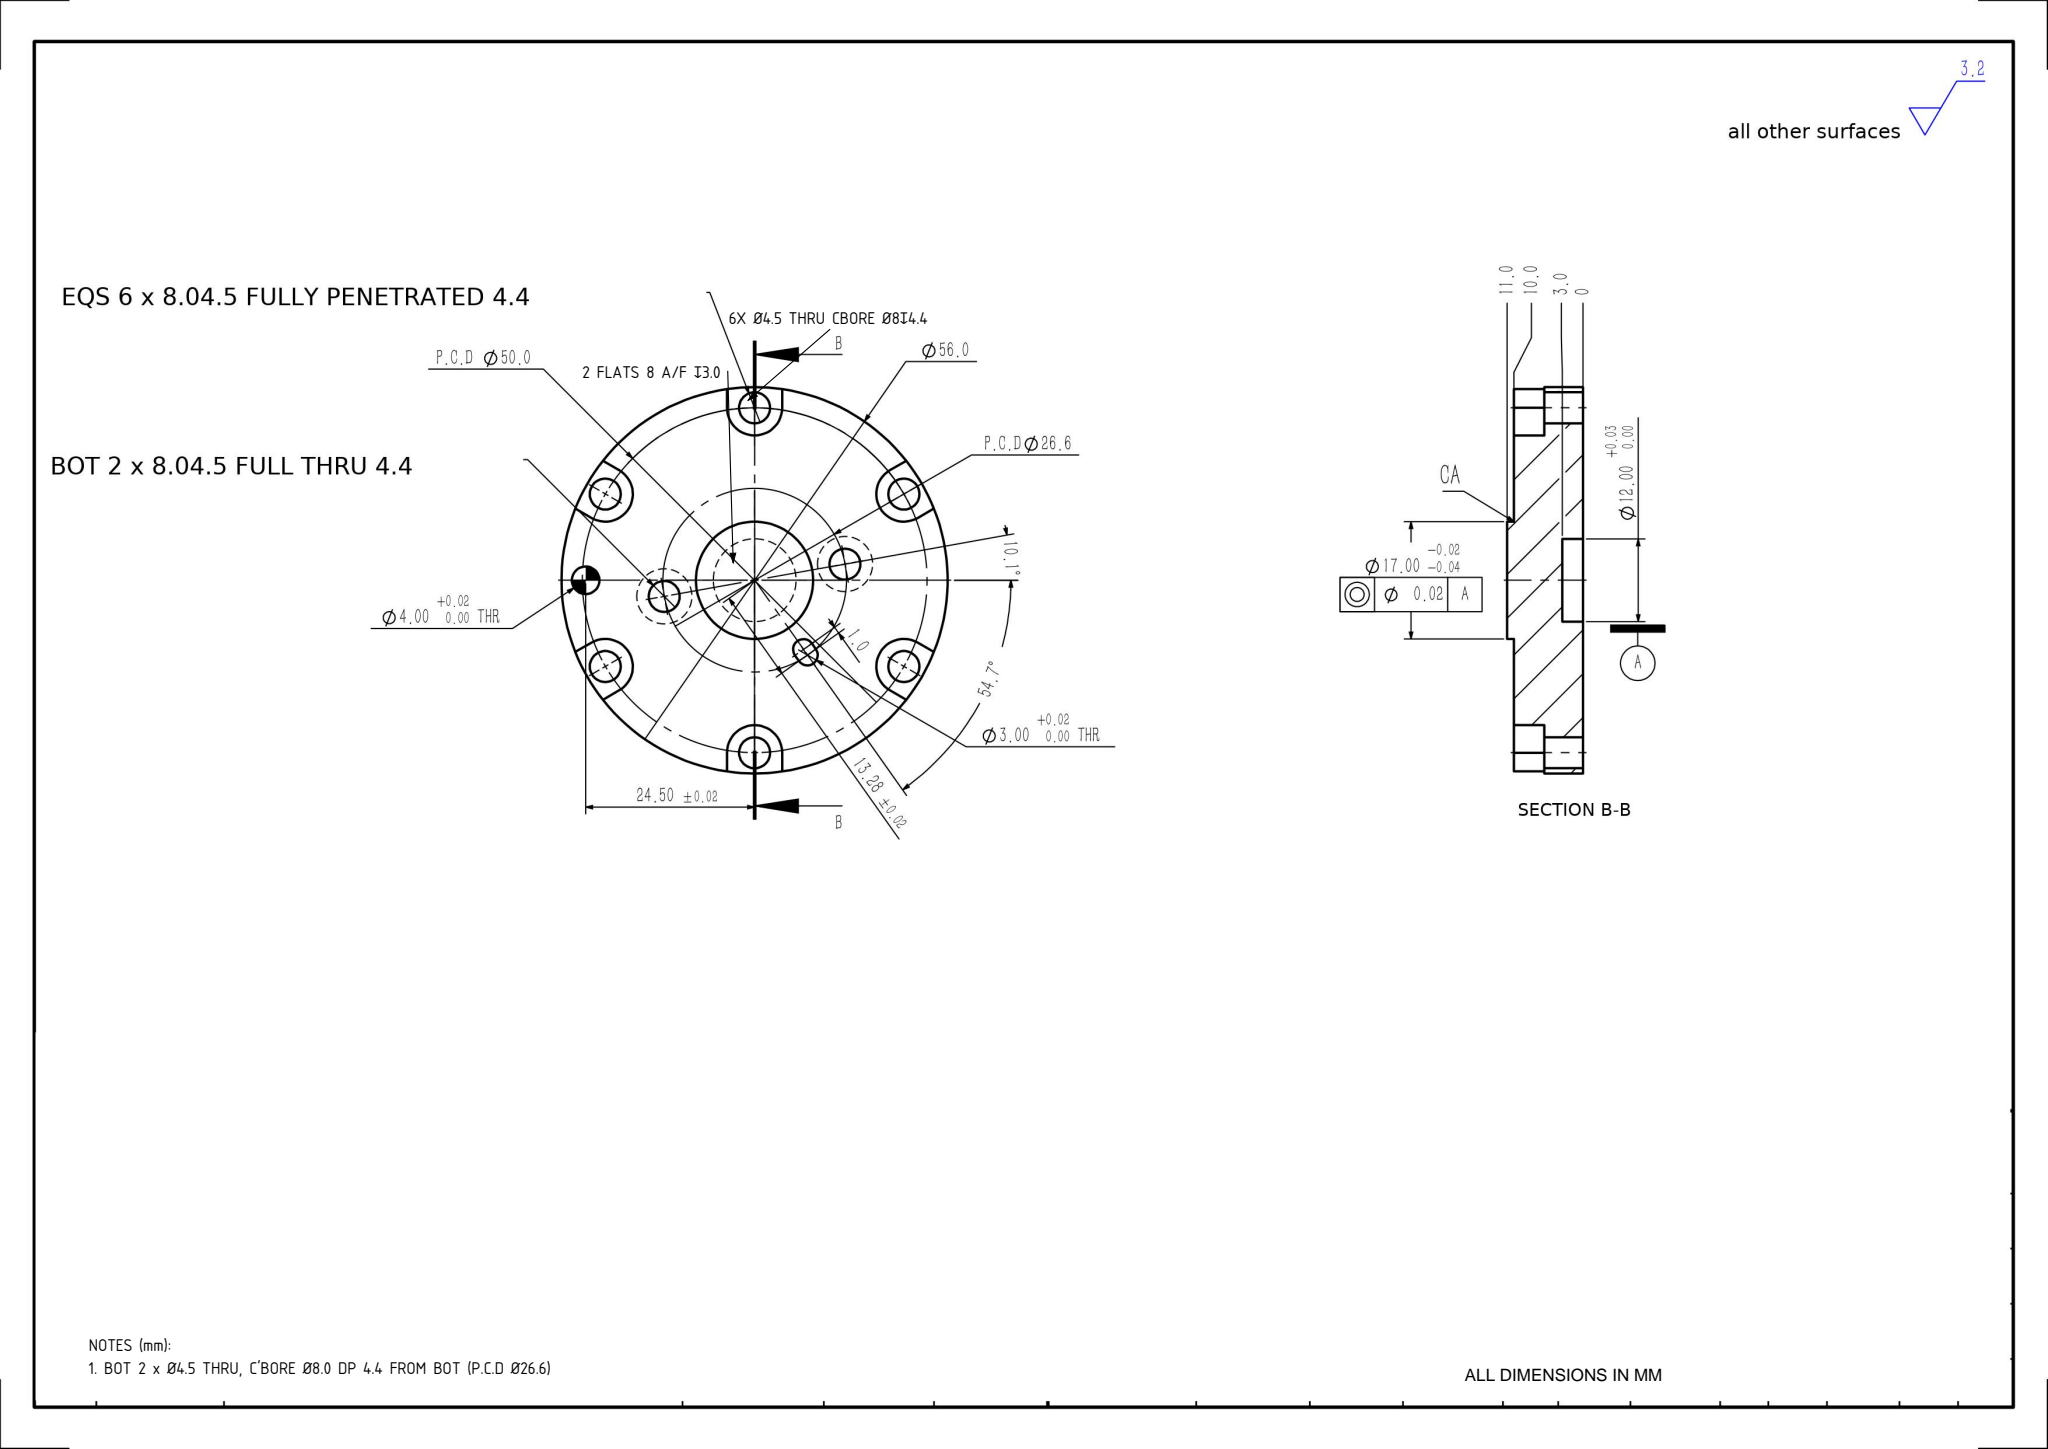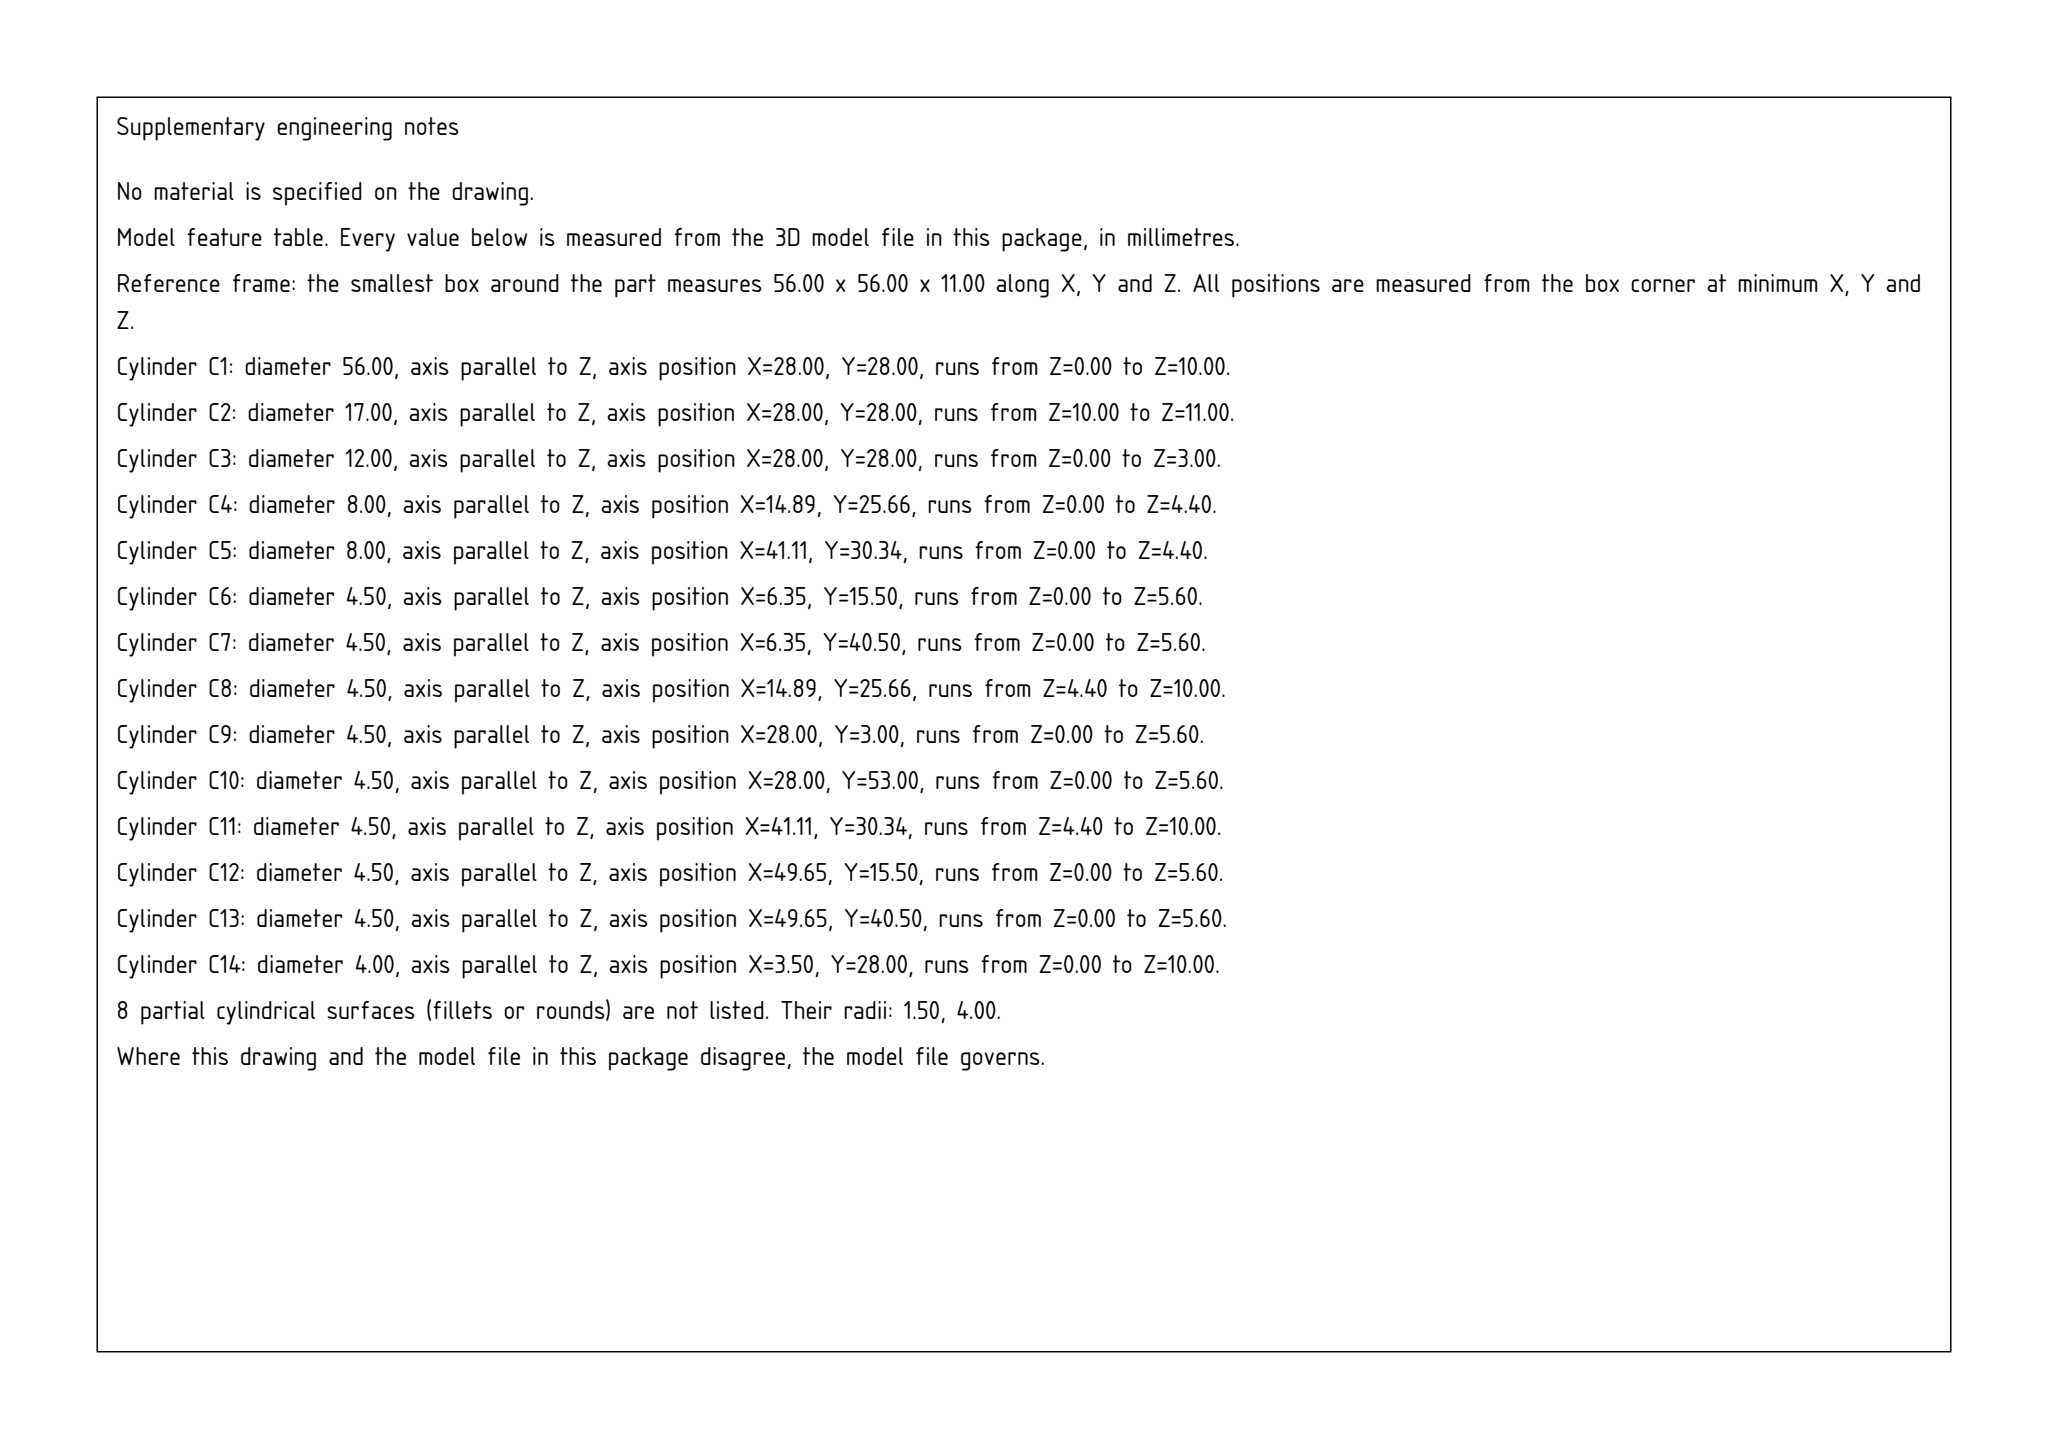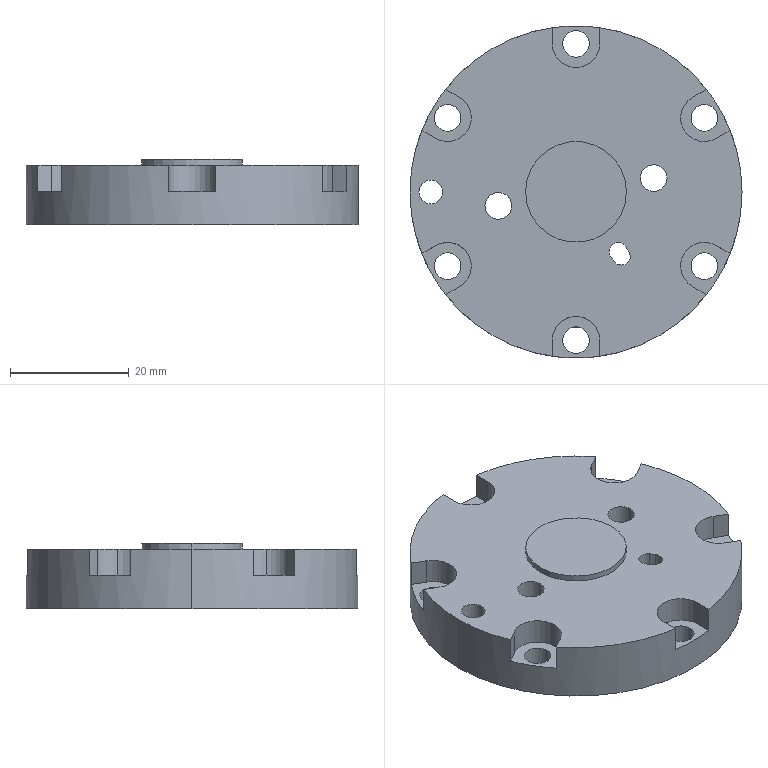Part | SolidWorks | mm | 1 solid | 65 faces | box 56 x 56 x 11 mm | volume 21860 mm3 | cylinder 39 | plane 26 | commonest cylinder face diameters 4.5 x16 8 x12 3 x3 4 x2 12 x2 17 x2 56 x2
Drawing notes:
2 FLATS 8.0 A/F SYM ABT AXIS ON Ø17 BOSS & Ø12 BORE, 3.0 DP | from the solid: axis_planes x=24.0 & x=32.0 (8.0 apart, sym about axis x=28.0) cutting Ø17.0 and Ø12.0 cyls at (28,28); Ø12 len 3.0
EQS 6 x Ø4.5 THRU, C'BORE Ø8.0 DP 4.4 (P.C.D Ø50.0) | from the solid: 6 cyl Ø4.5 len 5.6 + Ø8.0 len 4.4 at (6.35,15.5)(6.35,40.5)(28,3)(28,53)(49.65,15.5)(49.65,40.5), R25 from (28,28)
BOT 2 x Ø4.5 THRU, C'BORE Ø8.0 DP 4.4 FROM BOT (P.C.D Ø26.6) | from the solid: 2 cyl Ø4.5 len 5.6 + Ø8.0 len 4.4 at (14.89,25.66) & (41.11,30.34), R13.3 from (28,28)
build123d program:
from build123d import *

# Parameters (mm, degrees)
SKETCH1_R                                       = 28
BOSS_EXTRUDE1_DEPTH                             = 5.5
SKETCH2_R                                       = 28
SKETCH2_R_2                                     = 8.5
CUT_EXTRUDE1_DEPTH                              = 1
M4_HEX_SOCKET_HEAD_CAP_SCREW_CBORE2_D           = 4.5
M4_HEX_SOCKET_HEAD_CAP_SCREW_CBORE2_CBORE_D     = 8
M4_HEX_SOCKET_HEAD_CAP_SCREW_CBORE2_CBORE_DEPTH = 4.4
SKETCH8_W                                       = 8
SKETCH8_H                                       = 4
CUT_EXTRUDE2_DEPTH                              = 4.4
SKETCH9_R                                       = 6
CUT_EXTRUDE3_DEPTH                              = 3
SIZE_MM_DOWEL_PIN_HOLE1_D                       = 4
M4_HEX_SOCKET_HEAD_CAP_SCREW_CBORE3_D           = 4.5
M4_HEX_SOCKET_HEAD_CAP_SCREW_CBORE3_CBORE_D     = 8
M4_HEX_SOCKET_HEAD_CAP_SCREW_CBORE3_CBORE_DEPTH = 4.4
CUT_EXTRUDE5_DEPTH                              = 42.097


with BuildPart() as part:
    # Sketch1 → Boss-Extrude1 (new, symmetric)
    with BuildSketch(Plane.XY):
        Circle(SKETCH1_R)
    extrude(amount=BOSS_EXTRUDE1_DEPTH, both=True)

    # Sketch2 → Cut-Extrude1 (cut)
    with BuildSketch(Plane.XY.offset(5.5)):
        Circle(SKETCH2_R)
        Circle(SKETCH2_R_2, mode=Mode.SUBTRACT)
    extrude(amount=-CUT_EXTRUDE1_DEPTH, mode=Mode.SUBTRACT)

    # M4 Hex Socket Head Cap Screw CBORE2 (through all)
    with Locations(Plane.XY.offset(4.5)):
        with Locations((0, -25), (-21.651, -12.5), (-21.651, 12.5), (0, 25), (21.651, 12.5), (21.651, -12.5)):
            CounterBoreHole(M4_HEX_SOCKET_HEAD_CAP_SCREW_CBORE2_D / 2, M4_HEX_SOCKET_HEAD_CAP_SCREW_CBORE2_CBORE_D / 2, M4_HEX_SOCKET_HEAD_CAP_SCREW_CBORE2_CBORE_DEPTH)

    # Sketch8 → Cut-Extrude2 (cut)
    with BuildSketch(Plane.XY.offset(4.5)):
        Polygon((19.651, 15.964), (23.115, 17.964), (27.115, 11.036), (23.651, 9.036), align=None)
        with Locations((0, 27)):
            Rectangle(SKETCH8_W, SKETCH8_H)
        Polygon((23.651, -9.036), (27.115, -11.036), (23.115, -17.964), (19.651, -15.964), align=None)
        with Locations((0, -27)):
            Rectangle(SKETCH8_W, SKETCH8_H)
        Polygon((-19.651, -15.964), (-23.115, -17.964), (-27.115, -11.036), (-23.651, -9.036), align=None)
        Polygon((-23.651, 9.036), (-27.115, 11.036), (-23.115, 17.964), (-19.651, 15.964), align=None)
    extrude(amount=-CUT_EXTRUDE2_DEPTH, mode=Mode.SUBTRACT)

    # Sketch9 → Cut-Extrude3 (cut)
    with BuildSketch(Plane(origin=(0, 0, -5.5), x_dir=(-1, 0, 0), z_dir=(0, 0, -1))):
        Circle(SKETCH9_R)
    extrude(amount=-CUT_EXTRUDE3_DEPTH, mode=Mode.SUBTRACT)

    # Size mm Dowel Pin Hole1 (through all)
    with Locations(Plane.XY.offset(4.5)):
        with Locations((-24.5, 0)):
            Hole(SIZE_MM_DOWEL_PIN_HOLE1_D / 2)

    # M4 Hex Socket Head Cap Screw CBORE3 (through all)
    with Locations(Plane(origin=(0, 0, -5.5), x_dir=(-1, 0, 0), z_dir=(0, 0, -1))):
        with Locations((-13.106, 2.343), (13.106, -2.343)):
            CounterBoreHole(M4_HEX_SOCKET_HEAD_CAP_SCREW_CBORE3_D / 2, M4_HEX_SOCKET_HEAD_CAP_SCREW_CBORE3_CBORE_D / 2, M4_HEX_SOCKET_HEAD_CAP_SCREW_CBORE3_CBORE_DEPTH)

    # Sketch15 → Cut-Extrude5 (cut, through all)
    with BuildSketch(Plane(origin=(0, 0, -5.5), x_dir=(-1, 0, 0), z_dir=(0, 0, -1))):
        with BuildLine():
            Line((-8.891, -9.974), (-8.313, -9.157))
            ThreePointArc((-8.313, -9.157), (-6.223, -8.799), (-5.864, -10.89))
            Line((-5.864, -10.89), (-6.441, -11.706))
            ThreePointArc((-6.441, -11.706), (-8.532, -12.065), (-8.891, -9.974))
        make_face()
    extrude(amount=-CUT_EXTRUDE5_DEPTH, mode=Mode.SUBTRACT)


solid = part.part